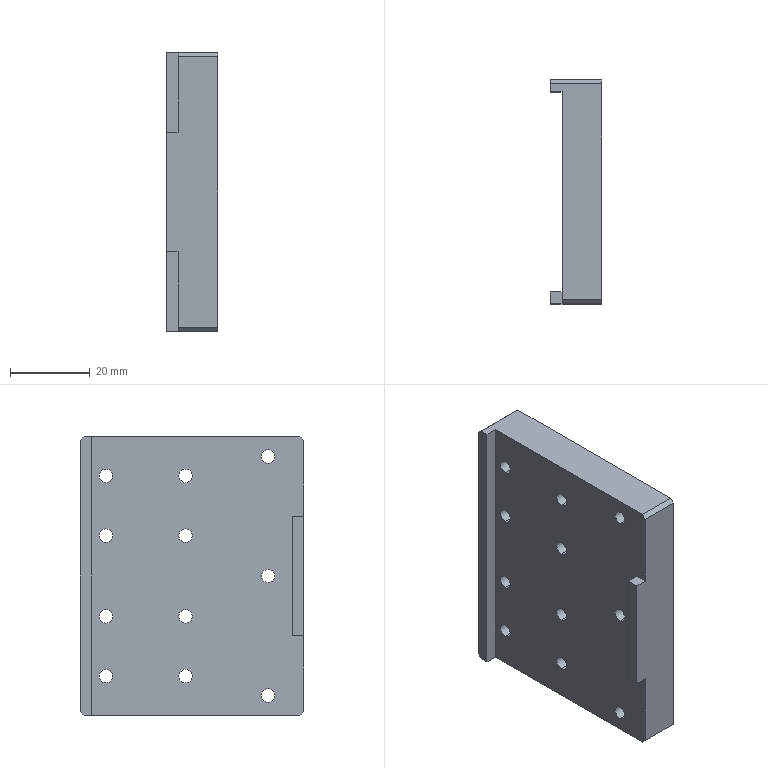Component | SolidWorks | F01AE00111-A2000-21TopEdgeAssembly-1_F01AE00111-A2051-1 | 1 solid | 83 faces | box 13 x 56.25 x 70 mm | volume 38384 mm3 | cylinder 50 | plane 27 | cone 6 | commonest cylinder face diameters 6 x22 3.4 x22 2.5 x6
build123d program:
from build123d import *

# Parameters (mm, degrees)
SKETCH1_W                                            = 70
SKETCH1_H                                            = 53.25
BOSS_EXTRUDE1_DEPTH                                  = 10
HOLE_SIZE_ACCORDING_TO_THE_TYPE_OF_HEXAG_D           = 3.4
HOLE_SIZE_ACCORDING_TO_THE_TYPE_OF_HEXAG_CBORE_D     = 6
HOLE_SIZE_ACCORDING_TO_THE_TYPE_OF_HEXAG_CBORE_DEPTH = 3.4
LPATTERN1_COUNT                                      = 3
LPATTERN1_PITCH                                      = 30
LPATTERN2_COUNT                                      = 3
LPATTERN2_PITCH                                      = 30
SKETCH8_W                                            = 13
SKETCH8_H                                            = 3
SKETCH8_W_2                                          = 3
BOSS_EXTRUDE2_DEPTH                                  = 70
HOLE_SIZE_ACCORDING_TO_THE_TYPE_OF_H_2_D             = 3.4
HOLE_SIZE_ACCORDING_TO_THE_TYPE_OF_H_2_CBORE_D       = 6
HOLE_SIZE_ACCORDING_TO_THE_TYPE_OF_H_2_CBORE_DEPTH   = 3.4
SKETCH12_W                                           = 20
SKETCH12_H                                           = 3
CUT_EXTRUDE1_DEPTH                                   = 10
CHAMFER1_SIZE                                        = 1


with BuildPart() as part:
    # Sketch1 → Boss-Extrude1 (new body)
    with BuildSketch(Plane.XY):
        Rectangle(SKETCH1_W, SKETCH1_H)
    extrude(amount=BOSS_EXTRUDE1_DEPTH)

    # Hole Size according to the type of hexag (through all)
    with Locations(Plane.XY.offset(10)):
        with Locations((-30, -20.625)):
            hole_size_according_to_the_type_of_hexag = CounterBoreHole(HOLE_SIZE_ACCORDING_TO_THE_TYPE_OF_HEXAG_D / 2, HOLE_SIZE_ACCORDING_TO_THE_TYPE_OF_HEXAG_CBORE_D / 2, HOLE_SIZE_ACCORDING_TO_THE_TYPE_OF_HEXAG_CBORE_DEPTH)

    # LPattern1: Hole Size according to the type of hexag ×3
    with Locations(*[(i * LPATTERN1_PITCH, 0, 0) for i in range(1, LPATTERN1_COUNT)]):
        add(hole_size_according_to_the_type_of_hexag, mode=Mode.SUBTRACT)

    # Sketch5 → M3 Tapped Hole1 (revolve, cut)
    with BuildSketch(Plane(origin=(-30, 26.625, 3), x_dir=(0, 0, 1), z_dir=(1, 0, 0))):
        Polygon((0, 0), (0, 10.751), (1.25, 10), (1.25, 0), align=None)
    m3_tapped_hole1 = revolve(axis=Axis((-30, 32.975, 3), (0, -1, 0)), mode=Mode.SUBTRACT)

    # LPattern2: M3 Tapped Hole1 ×3
    with Locations(*[(i * LPATTERN2_PITCH, 0, 0) for i in range(1, LPATTERN2_COUNT)]):
        add(m3_tapped_hole1, mode=Mode.SUBTRACT)

    # Sketch8 → Boss-Extrude2 (add)
    with BuildSketch(Plane.ZY.offset(35)):
        with Locations((3.5, -28.125)):
            Rectangle(SKETCH8_W, SKETCH8_H)
        with Locations((-1.5, 25.125)):
            Rectangle(SKETCH8_W_2, SKETCH8_H)
    extrude(amount=-BOSS_EXTRUDE2_DEPTH)

    # Hole Size according to the type of h 2 (through all)
    with Locations(Plane.XY.offset(10)):
        with Locations((-25.15, 20.125), (-25.15, 0.125), (-10.15, 0.125), (-10.15, 20.125), (10.15, 20.125), (10.15, 0.125), (25.15, 0.125), (25.15, 20.125)):
            CounterBoreHole(HOLE_SIZE_ACCORDING_TO_THE_TYPE_OF_H_2_D / 2, HOLE_SIZE_ACCORDING_TO_THE_TYPE_OF_H_2_CBORE_D / 2, HOLE_SIZE_ACCORDING_TO_THE_TYPE_OF_H_2_CBORE_DEPTH)

    # Sketch12 → Cut-Extrude1 (cut)
    with BuildSketch(Plane.XZ.offset(29.625)):
        with Locations((-25, -1.5)):
            Rectangle(SKETCH12_W, SKETCH12_H)
        with Locations((25, -1.5)):
            Rectangle(SKETCH12_W, SKETCH12_H)
    extrude(amount=-CUT_EXTRUDE1_DEPTH, mode=Mode.SUBTRACT)

    # Chamfer1
    chamfer1_edges = [part.edges().sort_by_distance(p)[0] for p in [
        (35, 26.625, 3.5),
        (-35, 26.625, 3.5),
        (35, -29.625, 5),
        (-35, -29.625, 5),
    ]]
    chamfer(chamfer1_edges, length=CHAMFER1_SIZE)


solid = part.part

# Placed as in the assembly
solid = solid.moved(Location((-74.352, 72.173, -299.975), (0, 90, 0)))